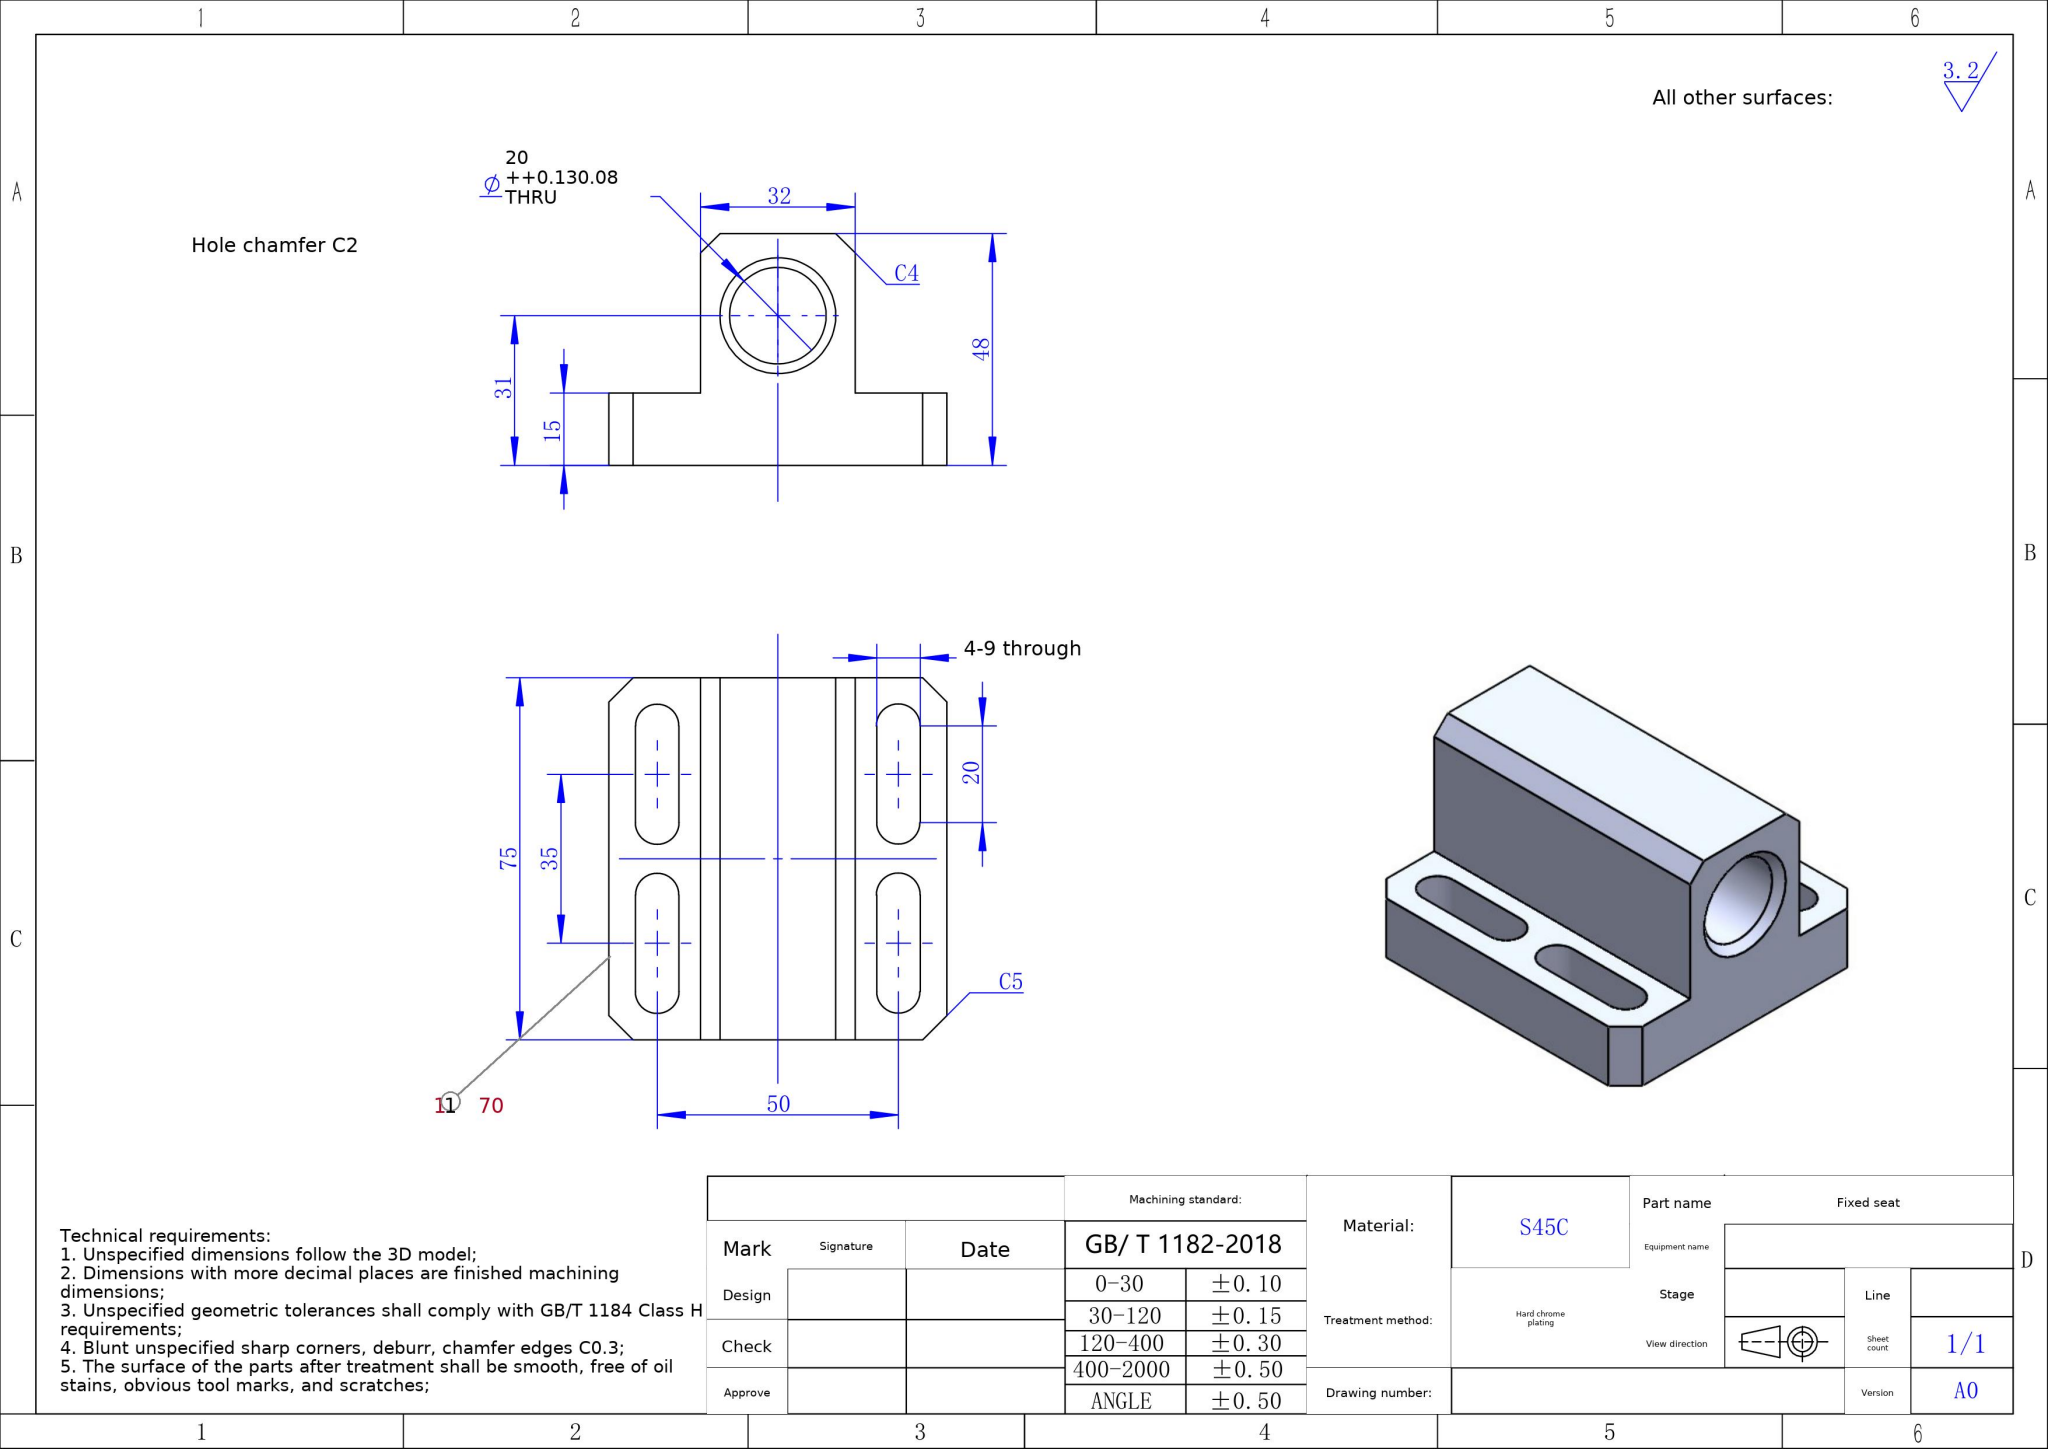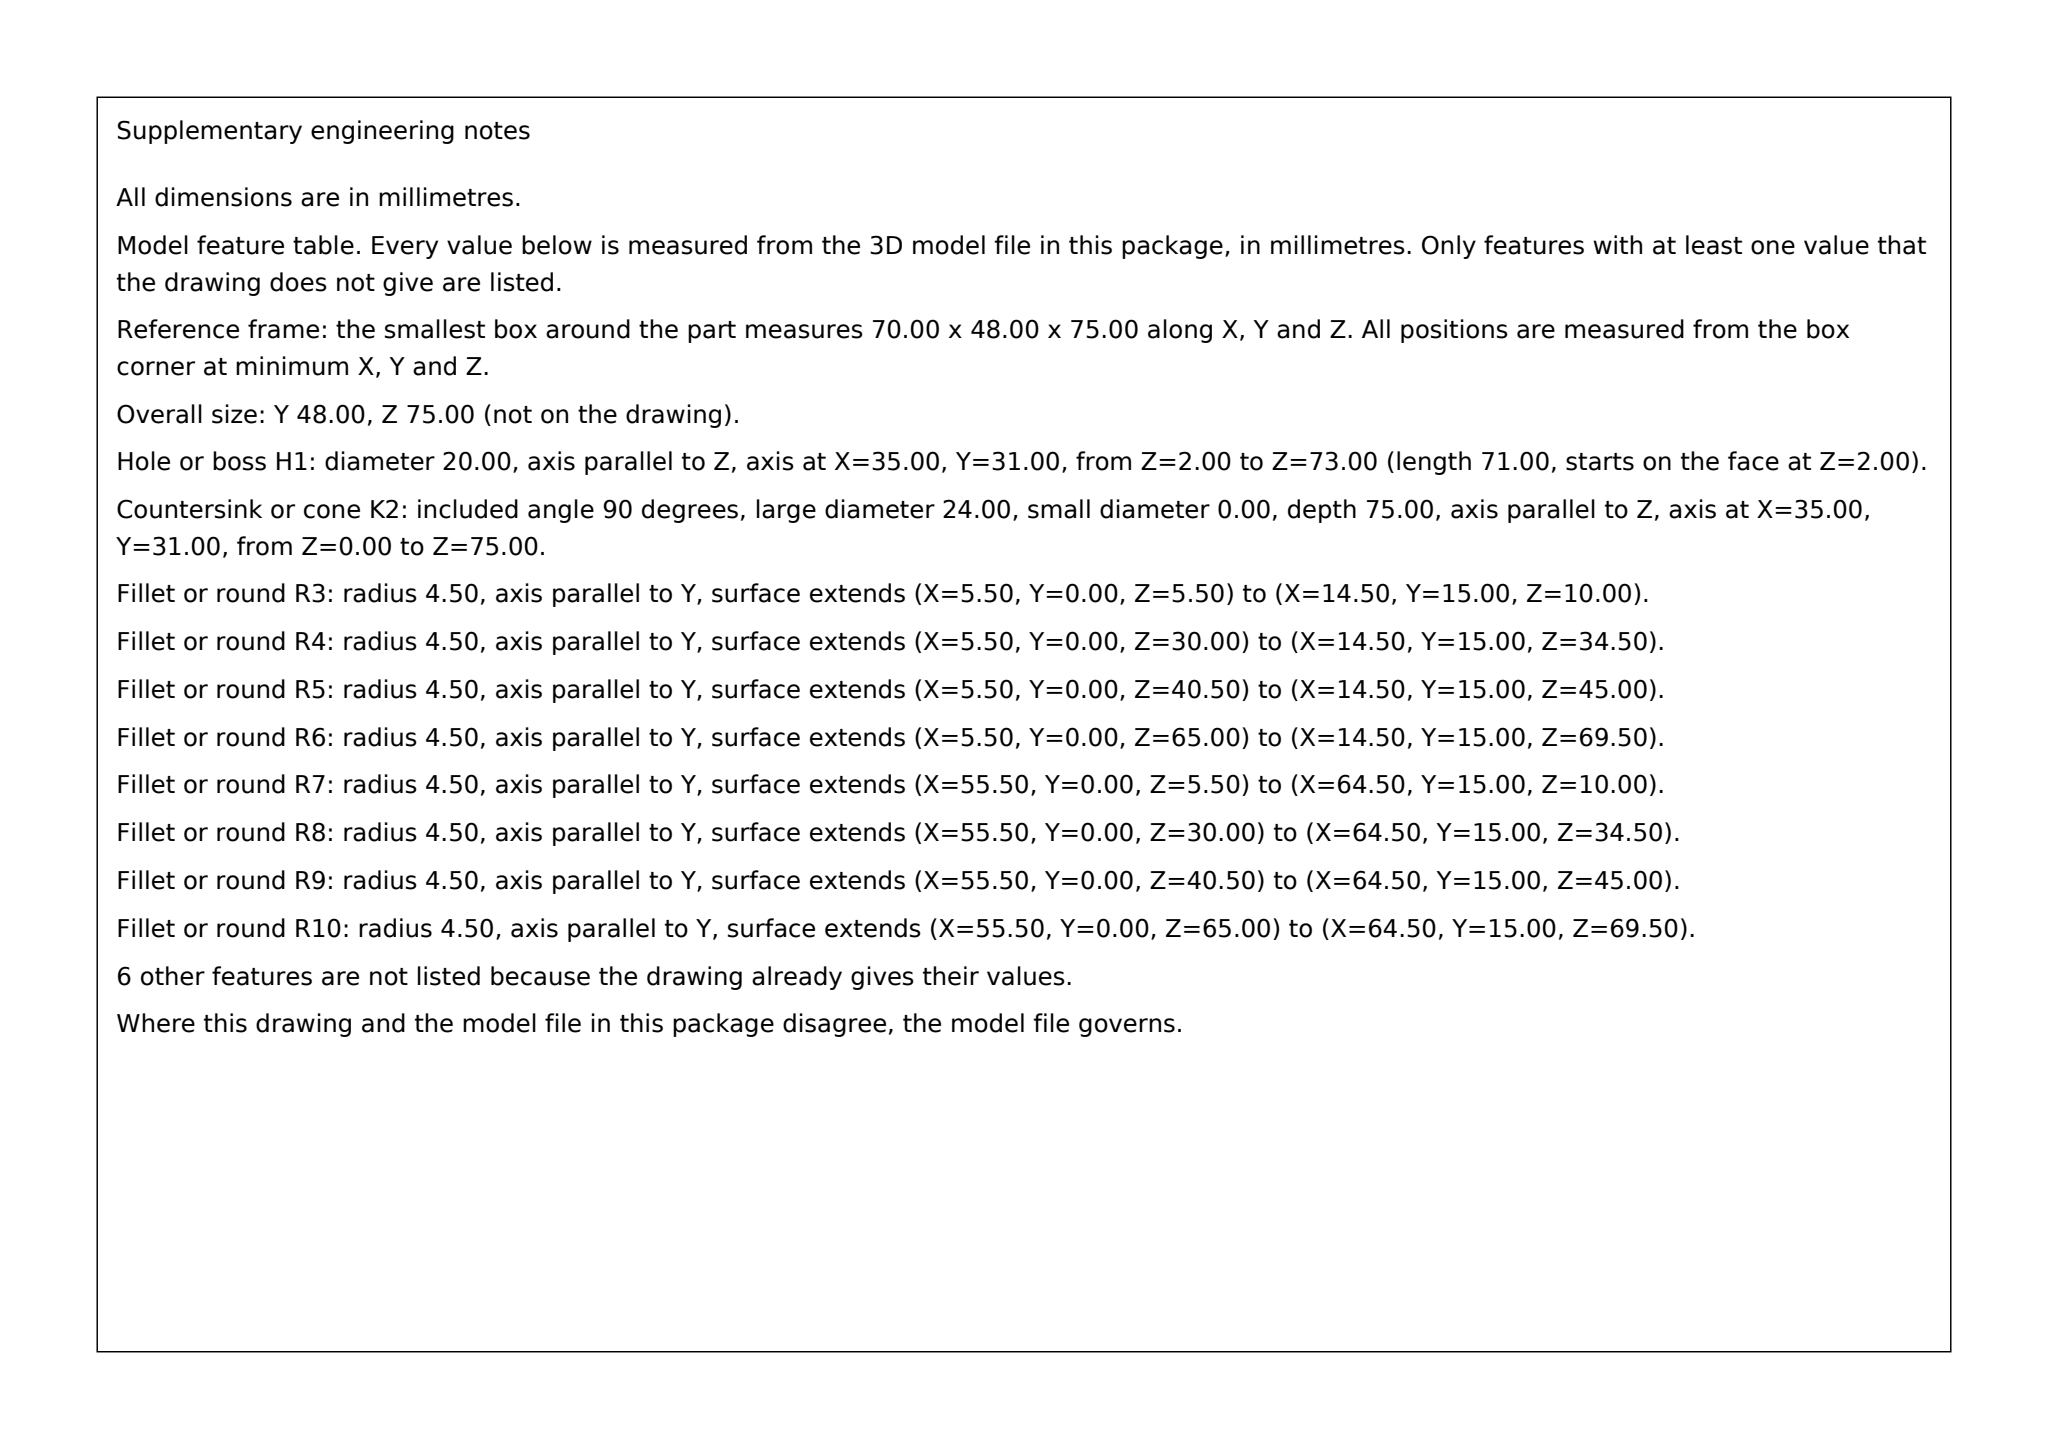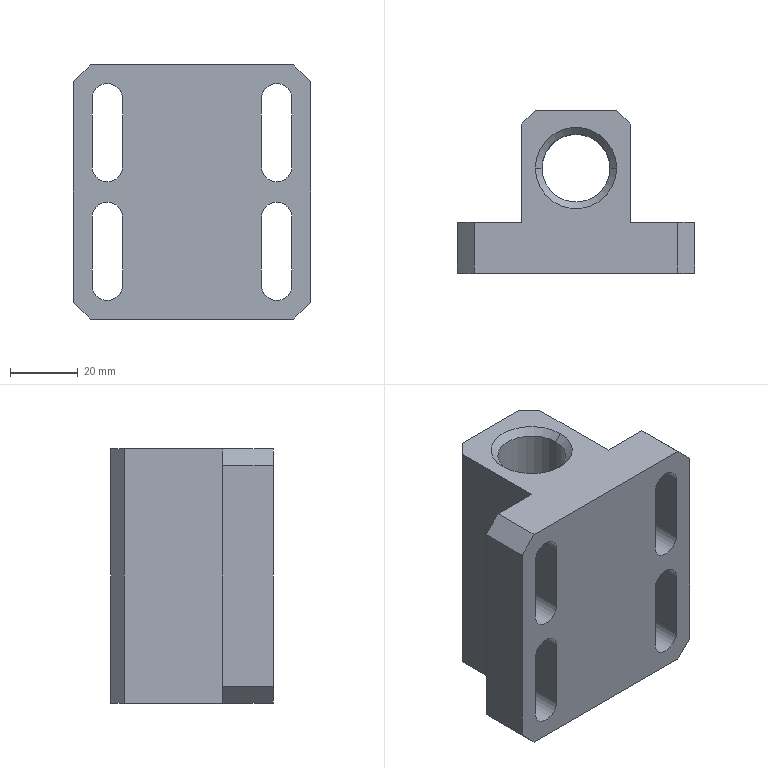Part | SolidWorks | mm | material S45C | 1 solid | 38 faces | box 70 x 48 x 75 mm | volume 117553 mm3 | plane 24 | cylinder 10 | cone 4 | commonest cylinder face diameters 9 x8 20 x2
build123d program:
from build123d import *

# Parameters (mm, degrees)
BOSS_EXTRUDE1_DEPTH = 37.5
CHAMFER1_SIZE       = 4
CHAMFER2_SIZE       = 5
SKETCH2_R           = 10
CUT_EXTRUDE1_DEPTH  = 96.677
CUT_EXTRUDE2_DEPTH  = 75
CHAMFER3_SIZE       = 2


with BuildPart() as part:
    # Sketch1 → Boss-Extrude1 (new, symmetric)
    with BuildSketch(Plane.XY):
        Polygon((-35, 0), (35, 0), (35, 15), (16, 15), (16, 48), (-16, 48), (-16, 15), (-35, 15), align=None)
    extrude(amount=BOSS_EXTRUDE1_DEPTH, both=True)

    # Chamfer1
    chamfer1_edges = [part.edges().sort_by_distance(p)[0] for p in [
        (-16, 48, 0),
        (16, 48, 0),
    ]]
    chamfer(chamfer1_edges, length=CHAMFER1_SIZE)

    # Chamfer2
    chamfer2_edges = [part.edges().sort_by_distance(p)[0] for p in [
        (35, 7.5, -37.5),
        (-35, 7.5, -37.5),
        (35, 7.5, 37.5),
        (-35, 7.5, 37.5),
    ]]
    chamfer(chamfer2_edges, length=CHAMFER2_SIZE)

    # Sketch2 → Cut-Extrude1 (cut, through all)
    with BuildSketch(Plane.XY.offset(37.5)):
        with Locations((0, 31)):
            Circle(SKETCH2_R)
    extrude(amount=-CUT_EXTRUDE1_DEPTH, mode=Mode.SUBTRACT)

    # Sketch3 → Cut-Extrude2 (cut)
    with BuildSketch(Plane(origin=(0, 15, 0), x_dir=(1, 0, 0), z_dir=(0, 1, 0))):
        with BuildLine():
            Line((29.5, 27.5), (29.5, 7.5))
            ThreePointArc((29.5, 7.5), (25, 3), (20.5, 7.5))
            Line((20.5, 7.5), (20.5, 27.5))
            ThreePointArc((20.5, 27.5), (25, 32), (29.5, 27.5))
        make_face()
        with BuildLine():
            Line((29.5, -27.5), (29.5, -7.5))
            ThreePointArc((29.5, -7.5), (25, -3), (20.5, -7.5))
            Line((20.5, -7.5), (20.5, -27.5))
            ThreePointArc((20.5, -27.5), (25, -32), (29.5, -27.5))
        make_face()
        with BuildLine():
            Line((-29.5, -27.5), (-29.5, -7.5))
            ThreePointArc((-29.5, -7.5), (-25, -3), (-20.5, -7.5))
            Line((-20.5, -7.5), (-20.5, -27.5))
            ThreePointArc((-20.5, -27.5), (-25, -32), (-29.5, -27.5))
        make_face()
        with BuildLine():
            Line((-29.5, 27.5), (-29.5, 7.5))
            ThreePointArc((-29.5, 7.5), (-25, 3), (-20.5, 7.5))
            Line((-20.5, 7.5), (-20.5, 27.5))
            ThreePointArc((-20.5, 27.5), (-25, 32), (-29.5, 27.5))
        make_face()
    extrude(amount=-CUT_EXTRUDE2_DEPTH, mode=Mode.SUBTRACT)

    # Chamfer3
    chamfer3_edges = [part.edges().sort_by_distance(p)[0] for p in [
        (-10, 31, -37.5),
        (-10, 31, 37.5),
    ]]
    chamfer(chamfer3_edges, length=CHAMFER3_SIZE)


solid = part.part